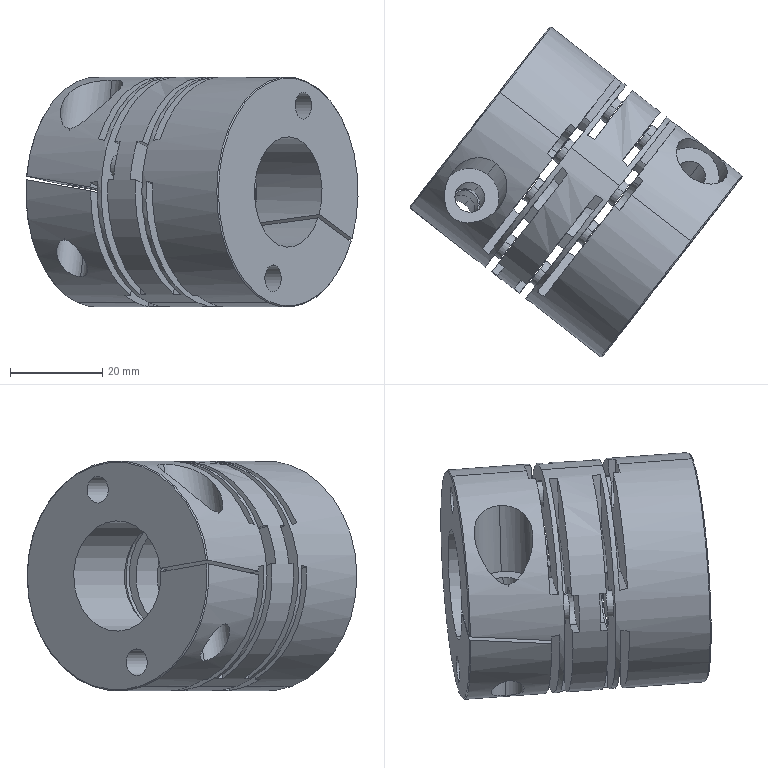Component | SolidWorks | MISUMI_MCSLC50-24-24_StandardCoupling-1_BODY_MISUMI_MCSLC50-24-24_StandardCoupling-1 | 1 solid | 154 faces | box 72.22 x 71.69 x 50 mm | volume 63004 mm3 | cylinder 78 | plane 70 | cone 6 | commonest cylinder face diameters 5.8 x24 8.5 x10 28 x10 24 x6 6 x5 6.6 x5 7.2 x4 12.75 x4